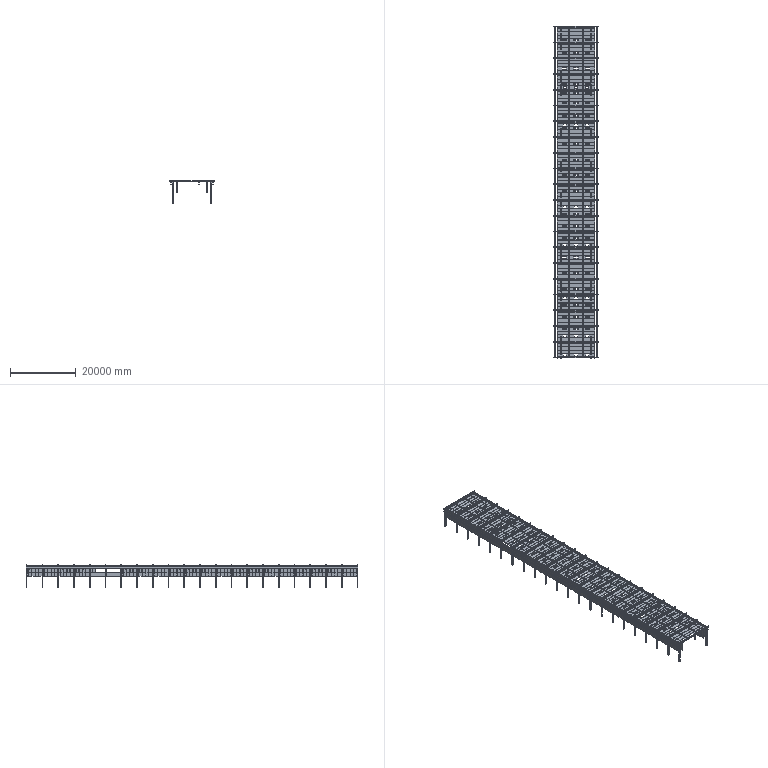Assembly | NX | mm | 1094 component files | 1134 solids | 18640 faces | box 13500 x 101200 x 6903 mm | volume 13637699093 mm3 | plane 17088 | cylinder 1516 | spline 36 | commonest cylinder face diameters 218 x608 20 x500 34 x246 27 x130 16 x28 200 x4
Bill of materials:
unnamed part 1 | 2 |  | Flat rectangular frame bent from round-section tube or rod, with rounded corners and two thinner straight crossbars running between the long sides.
unnamed part 2 | 1 |  | Long, narrow, thin rectangular flat plate or bar with no visible holes or cutouts.
unnamed part 3 | 2 |  | Long, slender, thin-walled member whose section is shown as Z-shaped: a central web with one leg turned up at one end and the other leg turned down at the other end.
unnamed part 4 | 56 |  | Thin rectangular flat plate, wider in proportion than a bar, with no visible holes or cutouts.
unnamed part 5 | 76 |  | Very thin rectangular sheet with four rounded corners and no visible holes.
unnamed part 6 | 1 |  | Thin rectangular flat plate with one elongated through slot (obround or rounded-rectangle) aligned with the long axis, set off-centre along the length.
unnamed part 7 | 2 |  | Long, slender, thin-walled round tube shown with a faceted (polygonal) circular section.
unnamed part 8 | 8 |  | Long, straight, solid bar with a rectangular cross-section.
unnamed part 9 | 22 |  | Long, straight beam with an I-shaped cross-section: two flat flanges joined by a thin central web.
unnamed part 10 | 3 |  | Very slender, long straight member with an I-shaped cross-section, with narrow flanges relative to its depth.
unnamed part 11 | 4 |  | Long, slender, thin-walled round tube with a faceted circular section, similar to the other tube in this set.
unnamed part 12 | 7 |  | Thin rectangular flat plate with one rectangular (near-square) through cutout near the middle of its length.
unnamed part 13 | 21 |  | Thin, elongated rectangular flat plate with a single rectangular through-cutout near the middle.
unnamed part 14 | 36 |  | Long, narrow, thin rectangular bar or strip with no visible holes or cutouts.
unnamed part 15 | 2 |  | Plain, long, narrow, thin rectangular plate with no visible openings.
unnamed part 16 | 2 |  | Long, slender, straight tube with a circular (faceted) annular cross-section.
unnamed part 17 | 2 |  | Long, slender, straight tube with a circular (faceted) annular cross-section; looks the same as unnamed part 16.
unnamed part 18 | 76 |  | Plain, thin, rectangular flat panel with no visible openings.
unnamed part 19 | 66 |  | Solid rectangular block (cuboid) with no visible holes or features.
unnamed part 20 | 2 |  | Long, slender, straight tube with a circular (faceted) annular cross-section; looks similar to the other tube parts.
unnamed part 21 | 82 |  | Thin rectangular flat panel with possible small edge features (chamfers or steps) along its two short ends.
unnamed part 22 | 4 |  | Very slender, straight thin-walled tube or rod with a circular (faceted) annular cross-section.
unnamed part 23 | 76 |  | Thin rectangular flat panel with one rounded-corner rectangular through-cutout in its upper portion, and possible edge features along the short ends.
unnamed part 24 | 112 |  | Plain, thin, elongated rectangular flat plate with no visible openings.
unnamed part 25 | 40 |  | Long, narrow, shallow rectangular tray: a flat rectangular base with a low, thin upturned rim along all four edges.
unnamed part 26 | 44 |  | Long straight lipped C-channel: a thin-walled open profile with a web, two parallel flanges and short return lips turned inward at the open side.
unnamed part 27 | 2 |  | Long, slender, straight hollow round tube with plain ends.
unnamed part 28 | 2 |  | Flat tubular frame: a rounded-corner rectangular loop of round tube with two thinner straight cross-bars spanning the shorter direction.
unnamed part 29 | 116 |  | Straight hollow round tube with two transverse cross holes spaced along its length and a shaped or angled feature at one end.
unnamed part 30 | 4 |  | Long, very slender, straight hollow round tube with plain ends.
unnamed part 31 | 2 |  | Long, slender, straight hollow round tube with plain ends.
unnamed part 32 | 4 |  | Long, slender, straight hollow round tube with plain ends.
unnamed part 33 | 2 |  | Long, slender, straight hollow round tube with plain ends.
unnamed part 34 | 22 |  | Very long, wide, shallow lipped channel: a thin-walled open profile with a wide web, short side walls and short inturned lips, plus one small notch or slot partway along its length.
unnamed part 35 | 41 |  | Shallow rectangular tray: a flat rectangular base with a low upturned rim on all edges, and one elongated rectangular through-cutout in the base, offset from center.
unnamed part 36 | 14 |  | Shallow rectangular tray: a flat rectangular base with a low upturned rim on all edges, and one large, nearly square rectangular through-cutout in the base, offset toward one end.
unnamed part 37 | 12 |  | Thin flat rectangular plate with one rectangular through-opening near one end.
unnamed part 38 | 4 |  | Very thin flat annular ring (washer-like) with a faceted, polygon-approximated circular outline.
unnamed part 39 | 2 |  | Plain thin flat rectangular plate with no visible features.
unnamed part 40 | 4 |  | Very thin flat annular ring with a faceted circular outline, nearly identical to the other ring parts.
unnamed part 41 | 2 |  | Long, thin-walled lipped C-channel: a web with two side flanges, each ending in a short inward-turned lip.
unnamed part 42 | 4 |  | Very thin flat annular ring with a faceted circular outline.
unnamed part 43 | 4 |  | Flat rectangular strip or plate, long relative to its width, with no visible features.
unnamed part 44 | 44 |  | Long straight I/H-section member: two parallel flanges joined by a central web of uniform section.
unnamed part 45 | 2 |  | Solid rectangular bar or thick plate, long relative to its width and thickness, with no visible features.
unnamed part 46 | 20 |  | Long, shallow, open rectangular tray: a flat base with a low wall around all four edges.
unnamed part 47 | 36 |  | Long, thin, bent-sheet profile with a Z-like section: a central web with legs at opposite ends turned in opposite directions.
unnamed part 48 | 2 |  | Long, very thin-walled lipped channel: a web, two flanges, and short inward lips.
Mates:
1. touch align | DB1 8 face | DB2 89 face
2. touch align | DB1 8 face | DB2 89 face
3. center | GD 3 face | GD 3 face | DB8 34 face | DB2 69 face
4. center | GDlianjie 65 face | GDlianjie 65 face | GD 3 face | GD 3 face
5. touch align | DS4 2 face | DS1 81 face
6. touch align | DS4 1 face | DS1 33 face